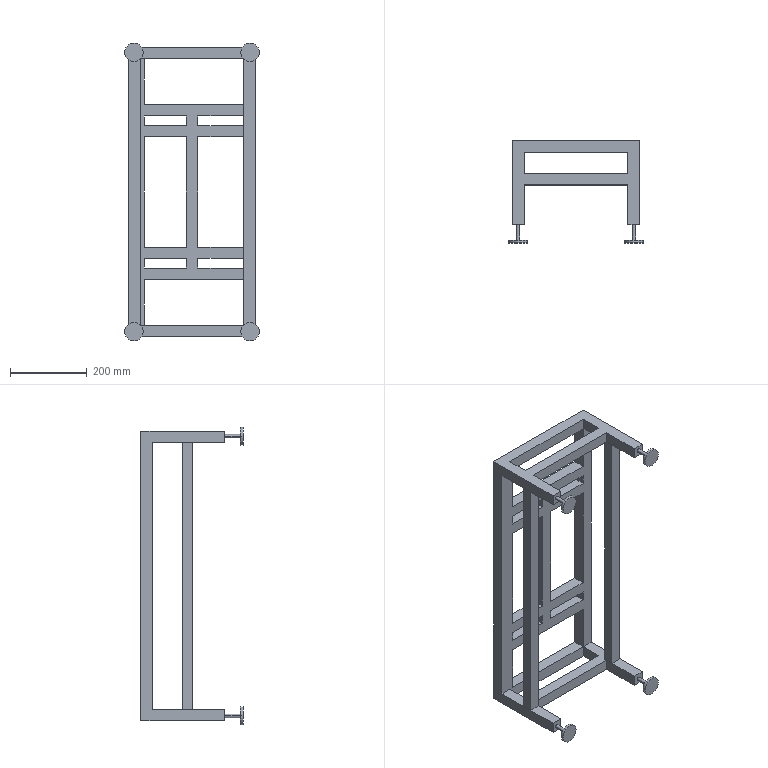Component | SolidWorks | Frame-1 | 3 solids | 92 faces | box 351.7 x 267 x 778.86 mm | volume 5558164 mm3 | plane 76 | cylinder 16 | commonest cylinder face diameters 48.35 x8 9.315 x8
build123d program:
from build123d import *

# Parameters (mm, degrees)
SKETCH1_W           = 330
SKETCH1_H           = 30
SKETCH1_W_2         = 30
SKETCH1_H_2         = 697.602
BOSS_EXTRUDE1_DEPTH = 30
BOSS_EXTRUDE4_DEPTH = 30
SKETCH3_W           = 29.256
SKETCH3_H           = 29.256
BOSS_EXTRUDE5_DEPTH = 189
SKETCH4_W           = 26.608
SKETCH4_H           = 699.09
BOSS_EXTRUDE6_DEPTH = 29.256
SKETCH5_W           = 271.488
SKETCH5_H           = 29.055
BOSS_EXTRUDE7_DEPTH = 29.256
SKETCH6_R           = 4.657
BOSS_EXTRUDE8_DEPTH = 41
SKETCH7_R           = 24.175
BOSS_EXTRUDE9_DEPTH = 7


with BuildPart() as part:
    # Sketch1 → Boss-Extrude1 (new body)
    with BuildSketch(Plane.XY):
        with Locations((0, -15)):
            Rectangle(SKETCH1_W, SKETCH1_H)
        Polygon((125, 0), (165, 0), (165, 697.602), (125, 697.602), (125, 348.801), align=None)
        with Locations((-150, 348.801)):
            Rectangle(SKETCH1_W_2, SKETCH1_H_2)
        with Locations((0, 712.602)):
            Rectangle(SKETCH1_W, SKETCH1_H)
    extrude(amount=BOSS_EXTRUDE1_DEPTH)

    # Sketch2 → Boss-Extrude4 (add)
    with BuildSketch(Plane.XY.offset(30)):
        Polygon((-135, 120.139), (125, 120.139), (125, 150.139), (15, 150.139), (15, 492.584), (125, 492.584), (125, 522.584), (-135, 522.584), (-135, 492.584), (-15, 492.584), (-15, 150.139), (-135, 150.139), align=None)
    extrude(amount=-BOSS_EXTRUDE4_DEPTH)

    # Sketch3 → Boss-Extrude5 (add)
    with BuildSketch(Plane.XY.offset(30)):
        with Locations((150.372, -15.372)):
            Rectangle(SKETCH3_W, SKETCH3_H)
        with Locations((-150.372, -15.372)):
            Rectangle(SKETCH3_W, SKETCH3_H)
        with Locations((-150.372, 712.974)):
            Rectangle(SKETCH3_W, SKETCH3_H)
        with Locations((150.372, 712.974)):
            Rectangle(SKETCH3_W, SKETCH3_H)
    extrude(amount=BOSS_EXTRUDE5_DEPTH)

    # Sketch5 → Boss-Extrude7 (add)
    with BuildSketch(Plane(origin=(0, 727.602, 0), x_dir=(1, 0, 0), z_dir=(0, 1, 0))):
        with Locations((0, -101.295)):
            Rectangle(SKETCH5_W, SKETCH5_H)
    extrude(amount=-BOSS_EXTRUDE7_DEPTH)


with BuildPart() as body_2:
    # Sketch4 → Boss-Extrude6 (new body)
    with BuildSketch(Plane.ZY.offset(165)):
        with Locations((122.789, 348.801)):
            Rectangle(SKETCH4_W, SKETCH4_H)
    extrude(amount=-BOSS_EXTRUDE6_DEPTH)


with BuildPart() as body_3:
    # Mirror1: mirrored copy
    add(body_2.part.mirror(Plane(origin=(0, 0, 0), x_dir=(0, 0, 1), z_dir=(1, 0, 0))))


with BuildPart() as body_4:
    # Mirror2: mirrored copy
    add(part.part.mirror(Plane.ZX.offset(348.801)))


with BuildPart() as part_1:
    add(part.part)

    add(body_4.part)  # Boss-Extrude8 merges body 4
    # Sketch6 → Boss-Extrude8 (add)
    with BuildSketch(Plane.XY.offset(219)):
        with Locations((151.696, -16.452)):
            Circle(SKETCH6_R)
        with Locations(Location((-151.658, -16.452, 0), (0, 0, 180))):
            Circle(SKETCH6_R)
    extrude(amount=BOSS_EXTRUDE8_DEPTH)

    # Sketch7 → Boss-Extrude9 (add)
    with BuildSketch(Plane.XY.offset(260)):
        with Locations((151.696, -16.452)):
            Circle(SKETCH7_R)
        with Locations((-151.658, -16.452)):
            Circle(SKETCH7_R)
    extrude(amount=BOSS_EXTRUDE9_DEPTH)

    # Mirror3: part across plane


with BuildPart() as part_2:
    add(part_1.part)
    add(part_1.part.mirror(Plane.ZX.offset(348.801)))


solid = Compound([body_2.part, body_3.part, part_2.part])

# Placed as in the assembly
solid = solid.moved(Location((0, -295.035, 48), (90, 0, -180)))